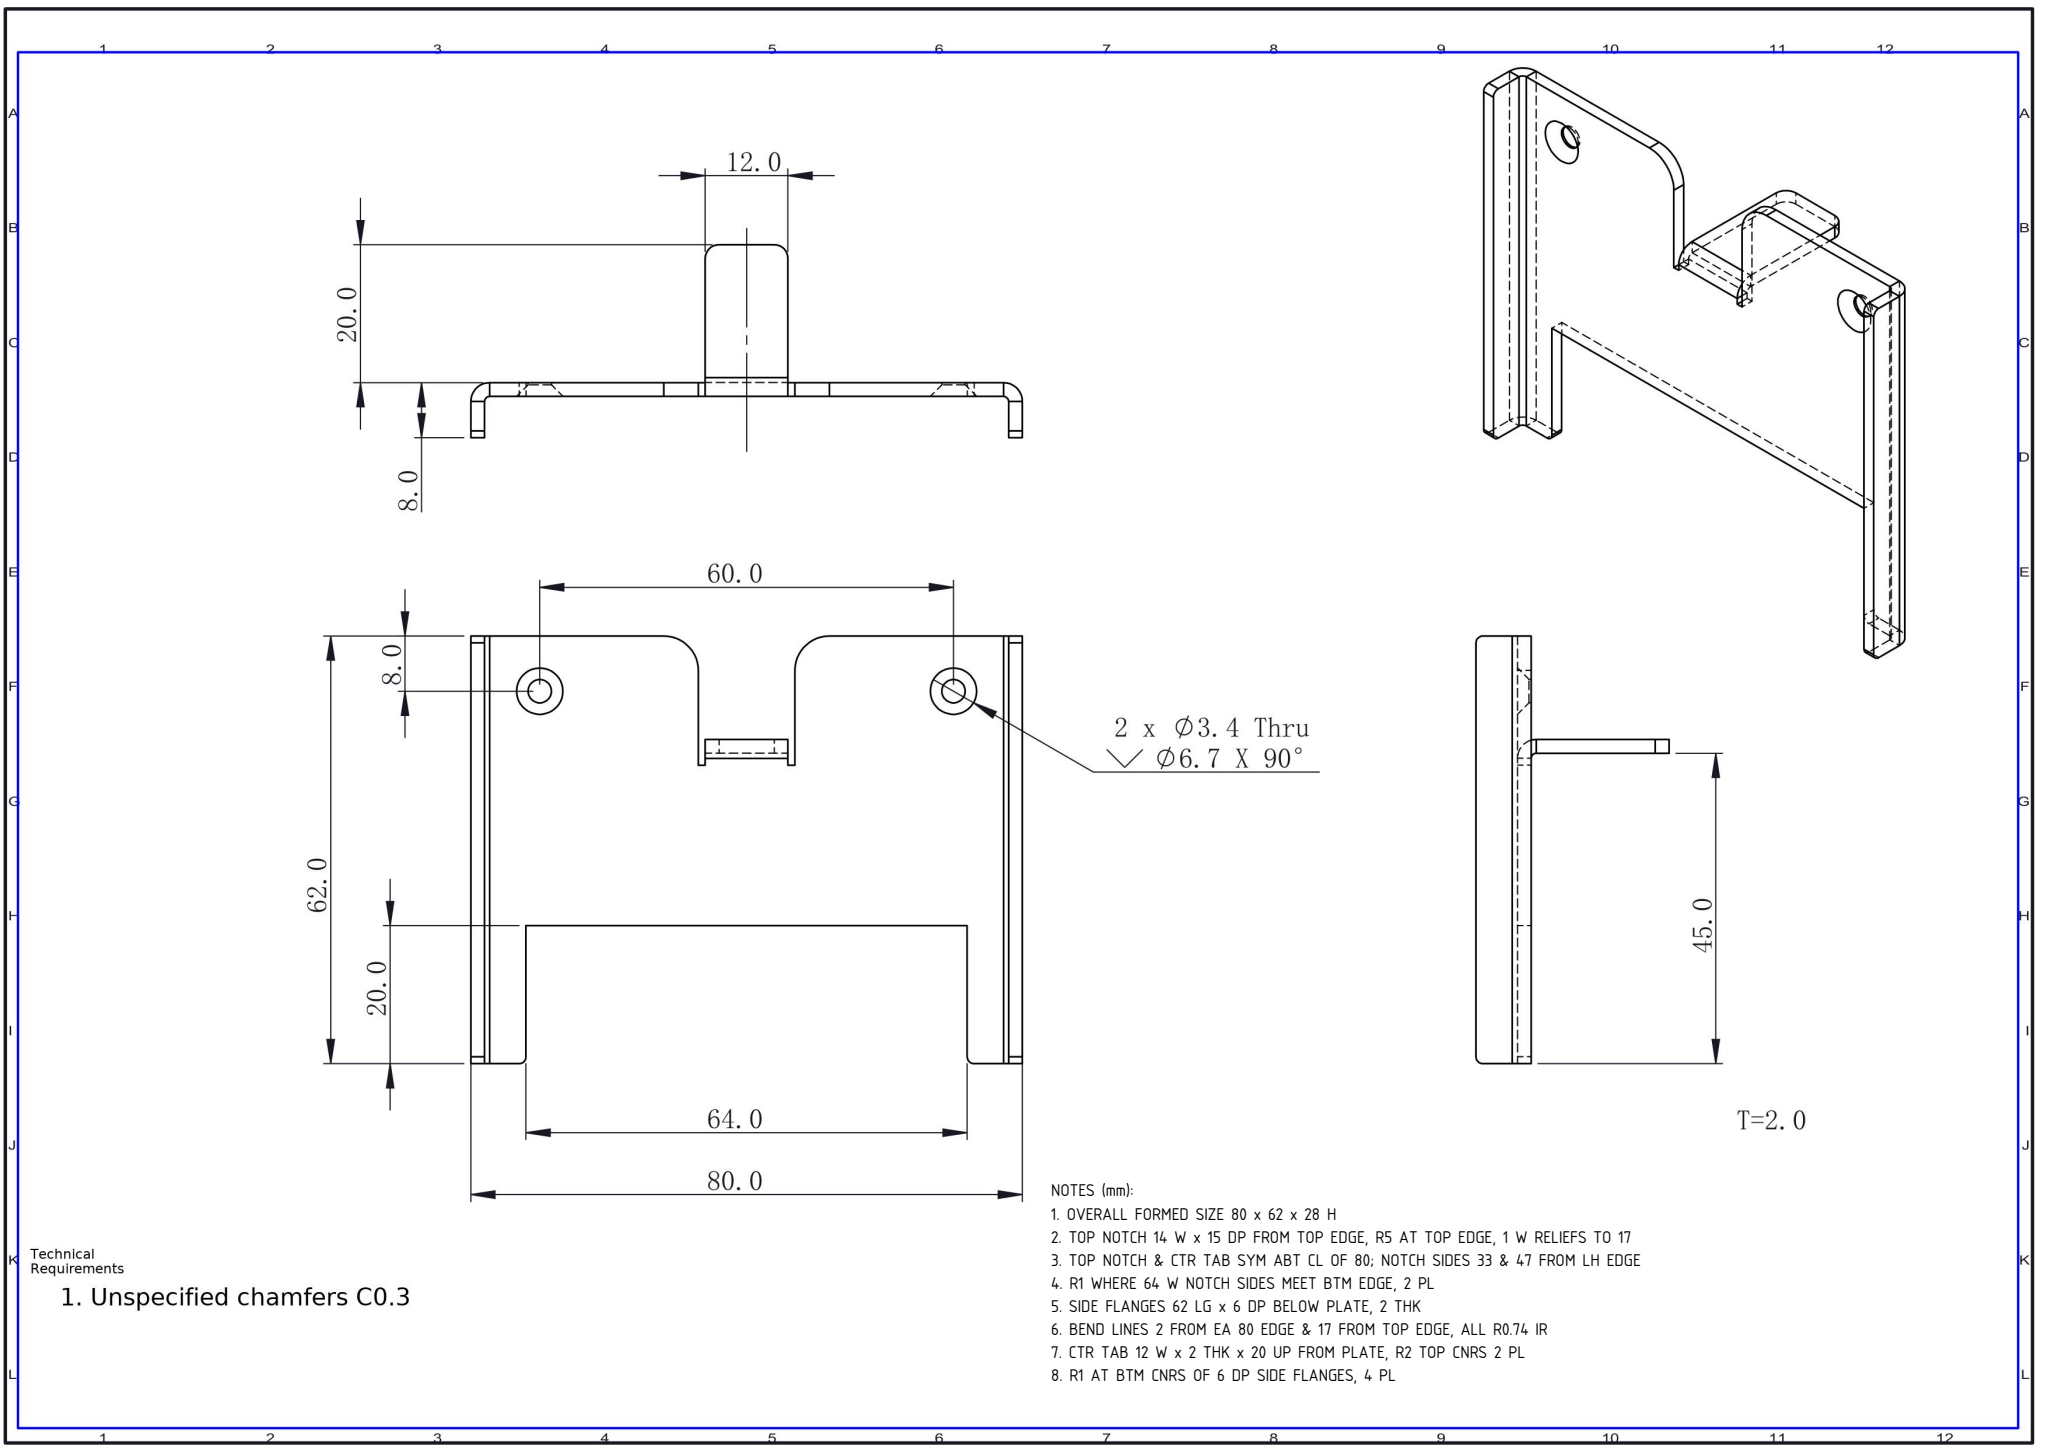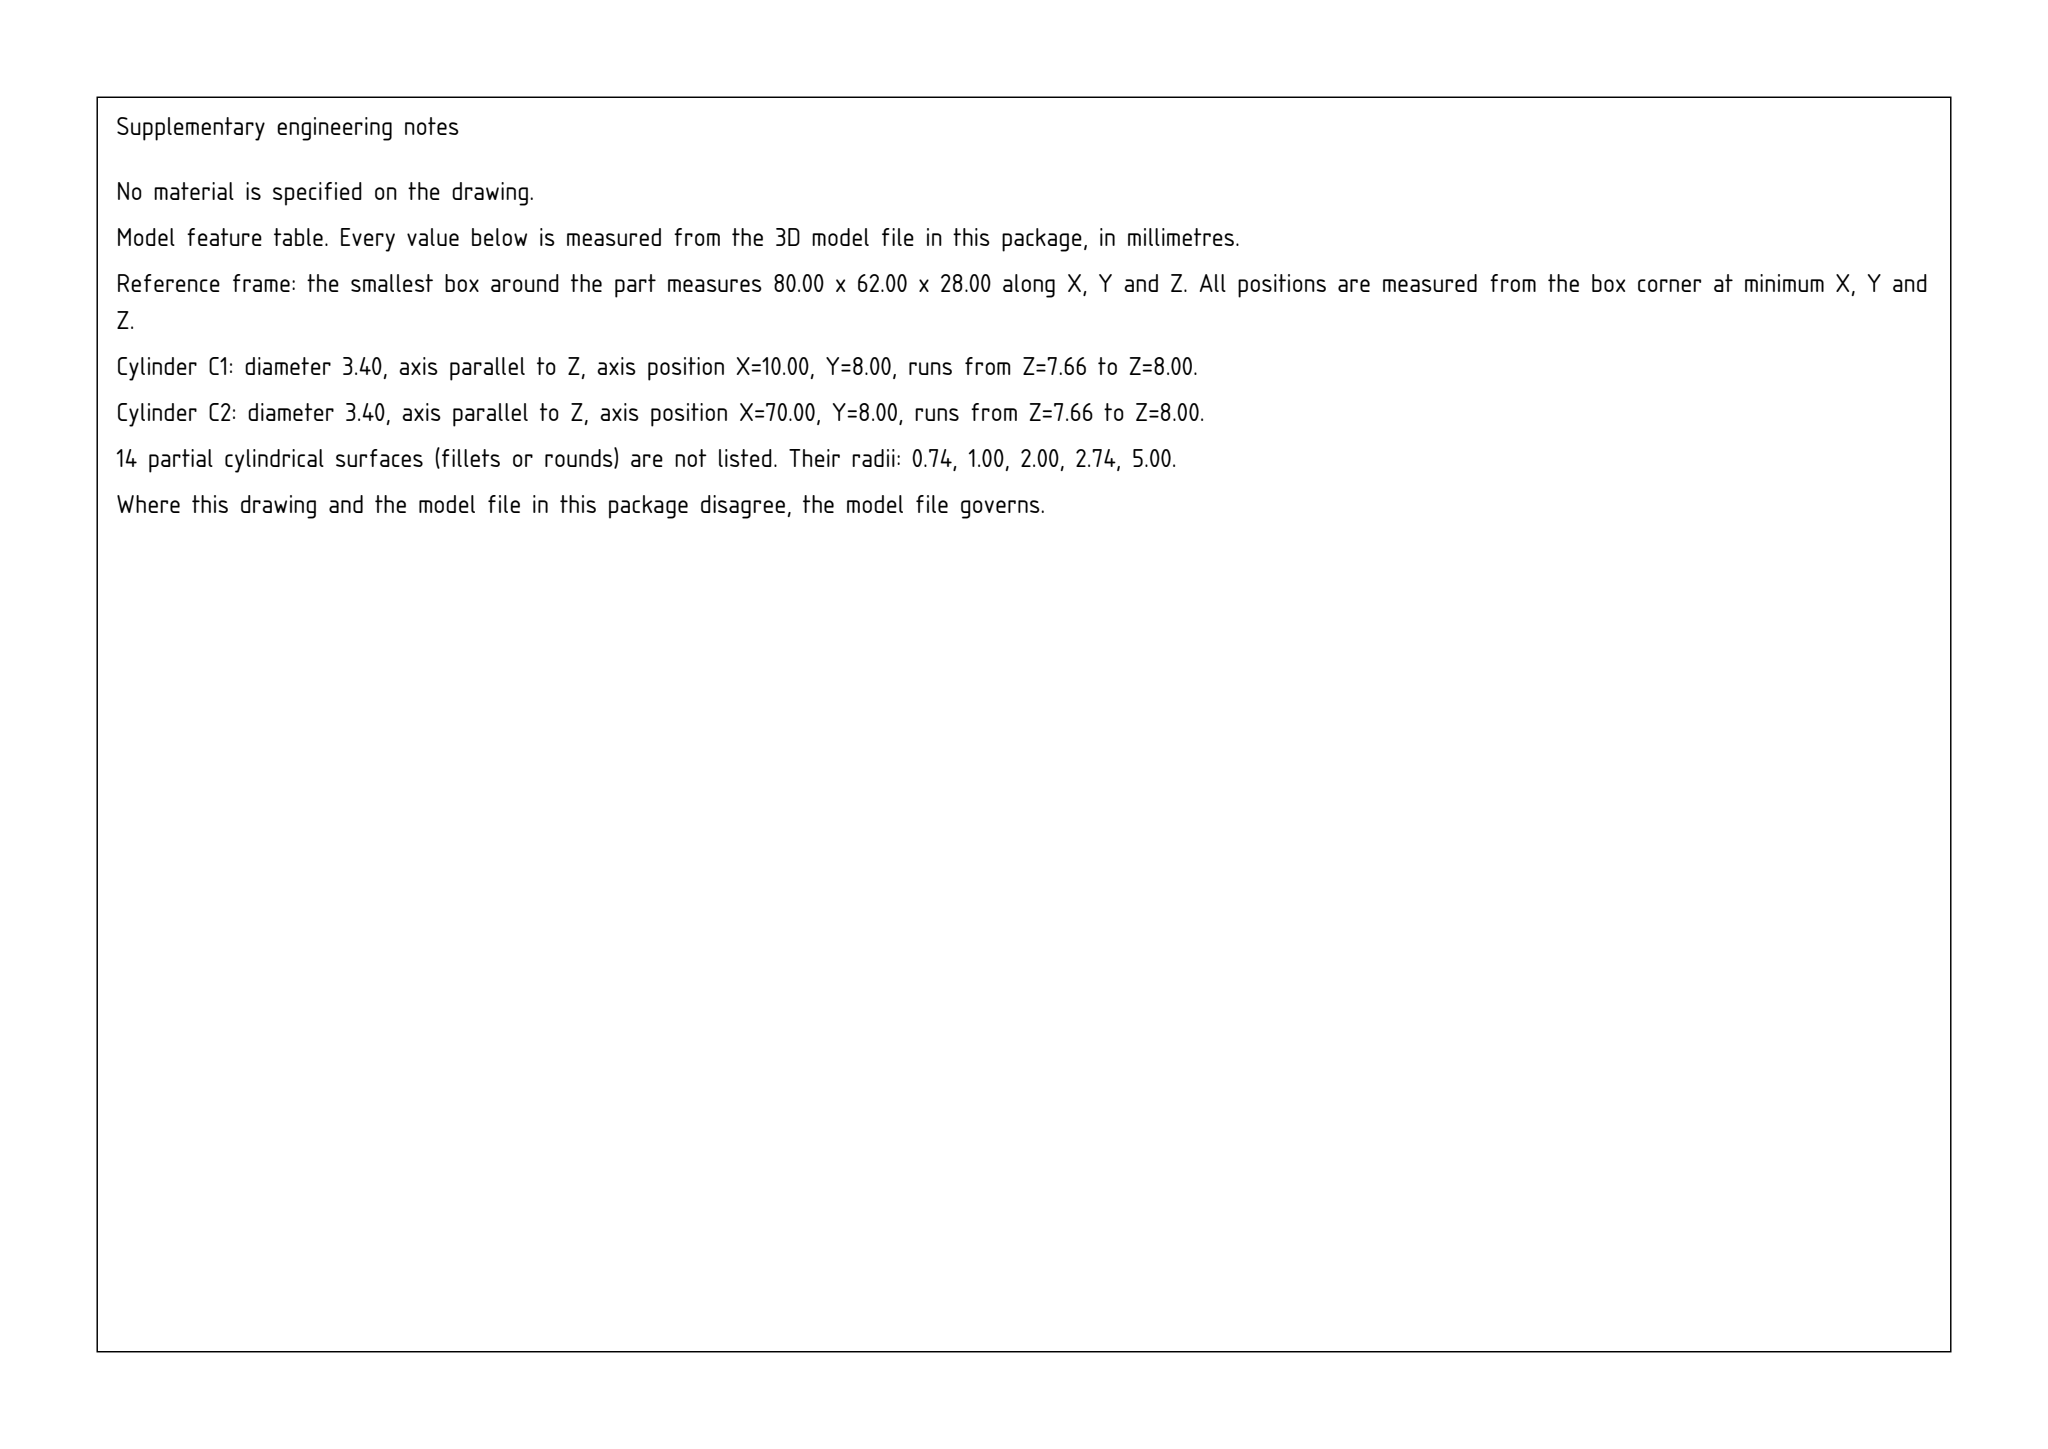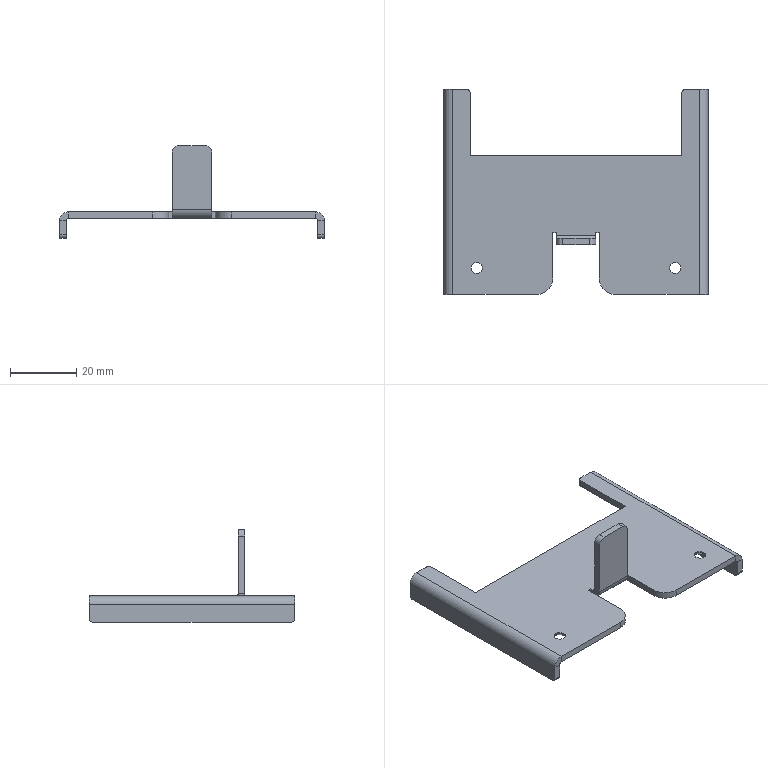Part | SolidWorks | mm | 1 solid | 60 faces | box 80 x 62 x 28 mm | volume 8588 mm3 | plane 36 | cylinder 20 | cone 4 | commonest cylinder face diameters 2 x6 3.4 x4 5.473 x3 1.473 x3 4 x2 10 x2
Drawing notes:
OVERALL FORMED SIZE 80 x 62 x 28 H | from the solid: bbox_xyz 80.0 x 62.0 x 28.0
TOP NOTCH 14 W x 15 DP FROM TOP EDGE, R5 AT TOP EDGE, 1 W RELIEFS TO 17 | from the solid: x-planes 33.0/47.0 = 14 W; y-plane 15.0 notch end; ø10 z-axis cyls at (28,5) & (52,5) = R5 tangent y=0; x-planes 34.0/46.0 reliefs to bend line y=17.0
TOP NOTCH & CTR TAB SYM ABT CL OF 80; NOTCH SIDES 33 & 47 FROM LH EDGE | from the solid: x-planes 33/47 midpoint 40 = 80/2; tab x 34-46 ctr 40
R1 WHERE 64 W NOTCH SIDES MEET BTM EDGE, 2 PL | from the solid: ø2.0 z-axis cyls at (7,61) & (73,61) lg 2.0 = plate thk; notch sides x8/x72, btm edge y62
SIDE FLANGES 62 LG x 6 DP BELOW PLATE, 2 THK | from the solid: y-axis bend cyls at x=2.74 & 77.26 lg 62.0; z-planes 0.0/6.0/8.0; faces x0/2.0 & 78.0/80.0
BEND LINES 2 FROM EA 80 EDGE & 17 FROM TOP EDGE, ALL R0.74 IR | from the solid: x-planes 2.0 & 78.0 flange inner faces; y-plane 17.0 tab face; bend cyls ø1.473 ID / ø5.473 OD
CTR TAB 12 W x 2 THK x 20 UP FROM PLATE, R2 TOP CNRS 2 PL | from the solid: tab x 34-46 = 12; y 15-17 = 2 thk; z 8-28 = 20; ø4.0 y-axis cyls at (36,26) & (44,26) lg 2.0
R1 AT BTM CNRS OF 6 DP SIDE FLANGES, 4 PL | from the solid: ø2.0 x-axis cyls at (y1,z1) & (y61,z1), 2 ea; flange btm z0, ends y0/y62